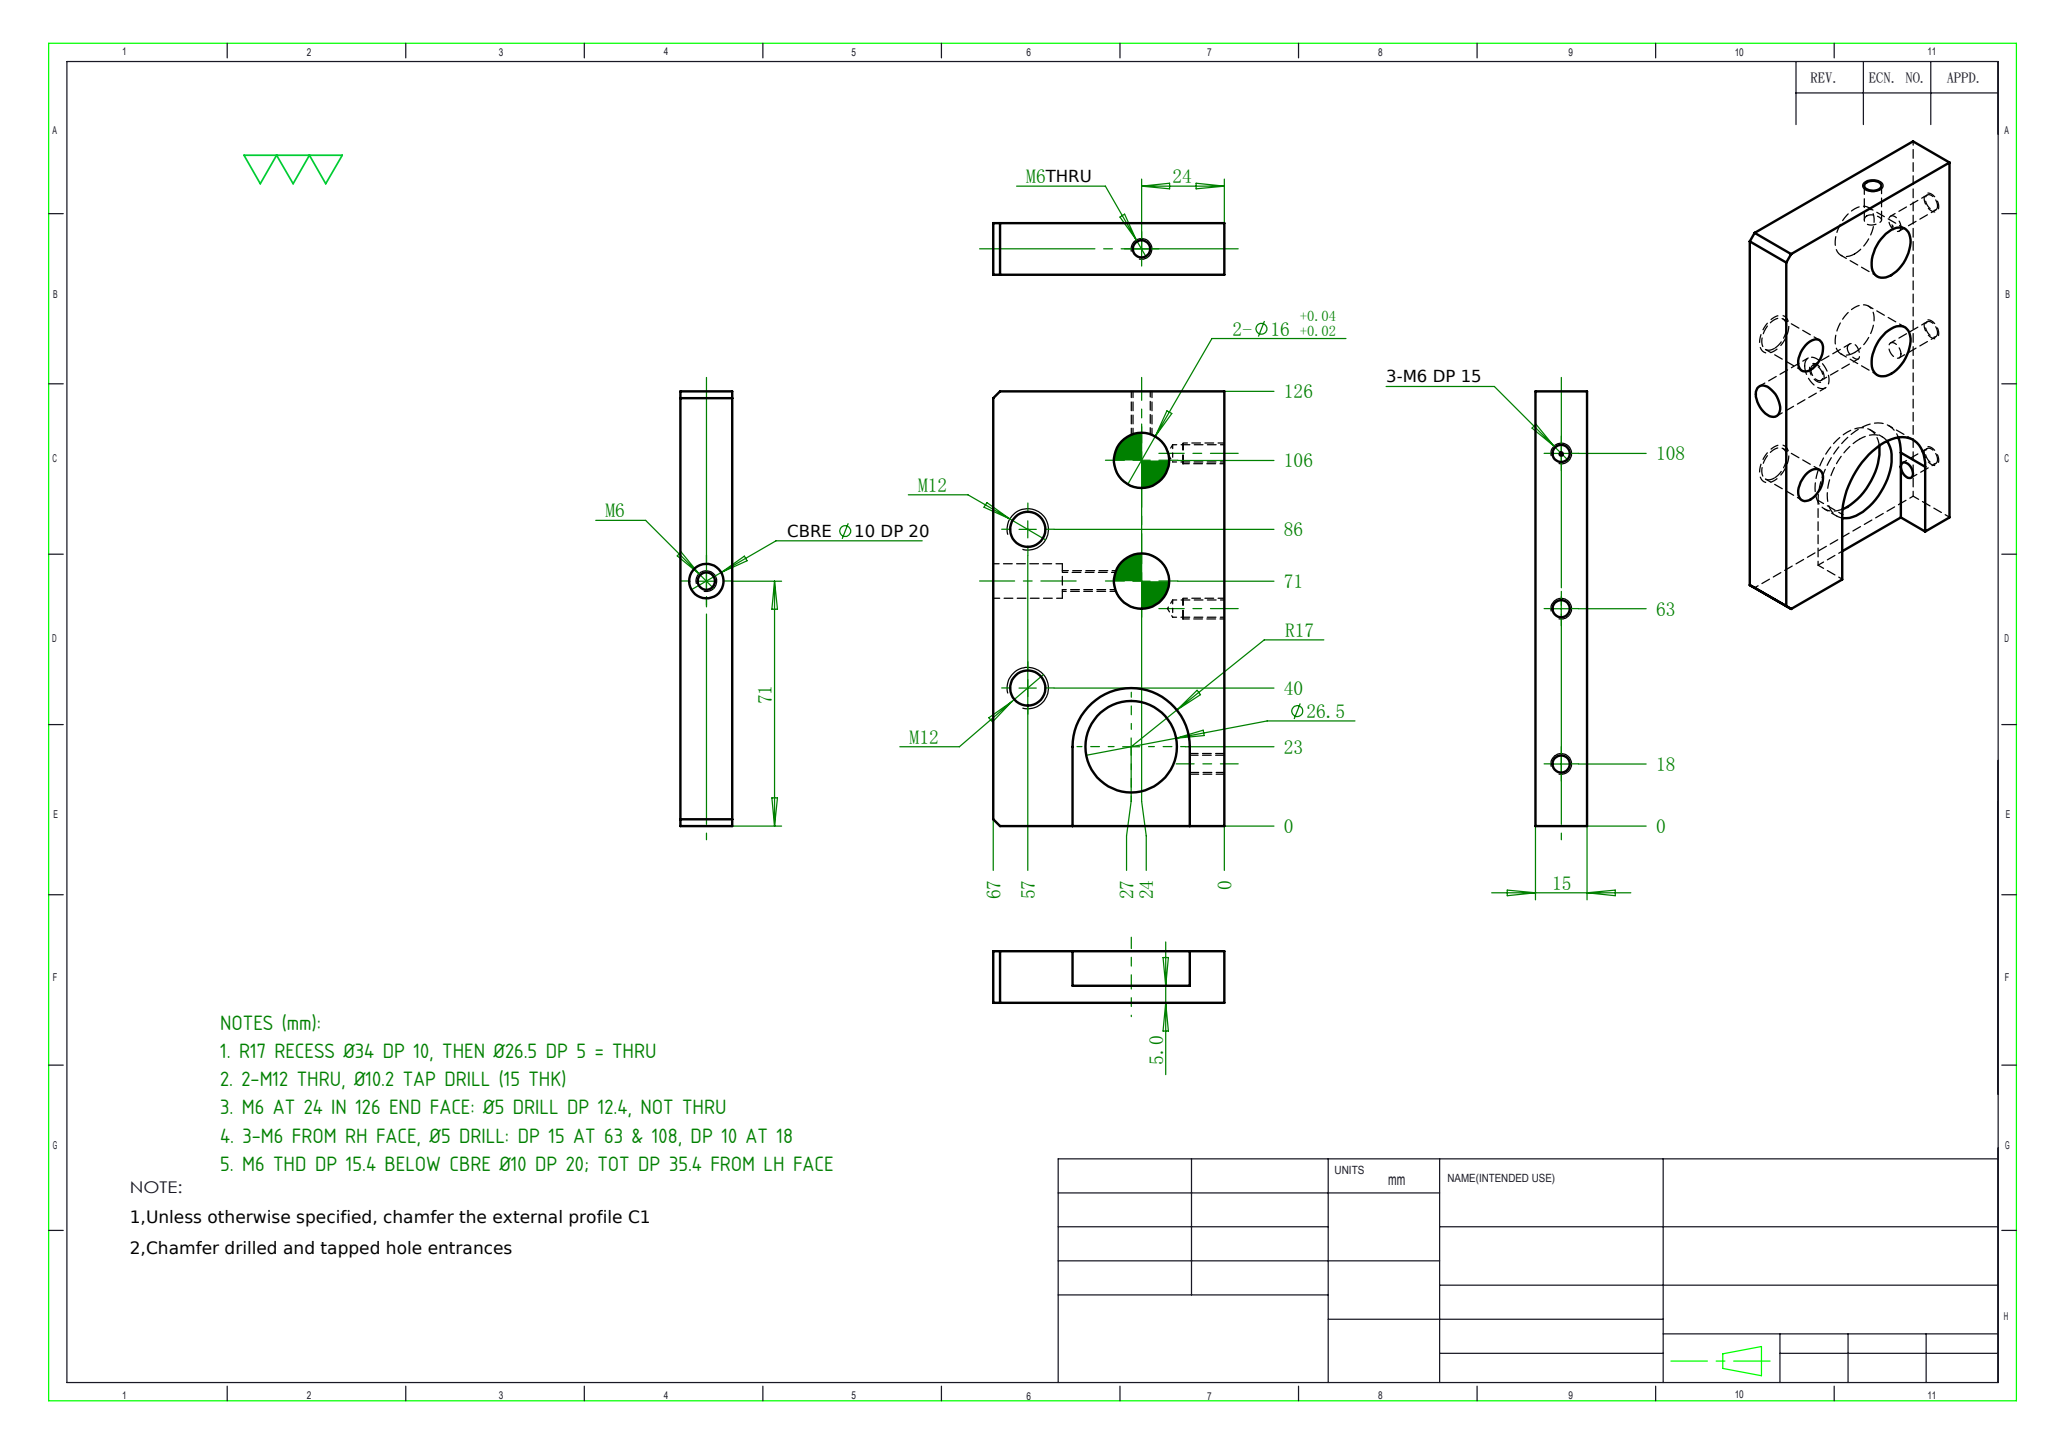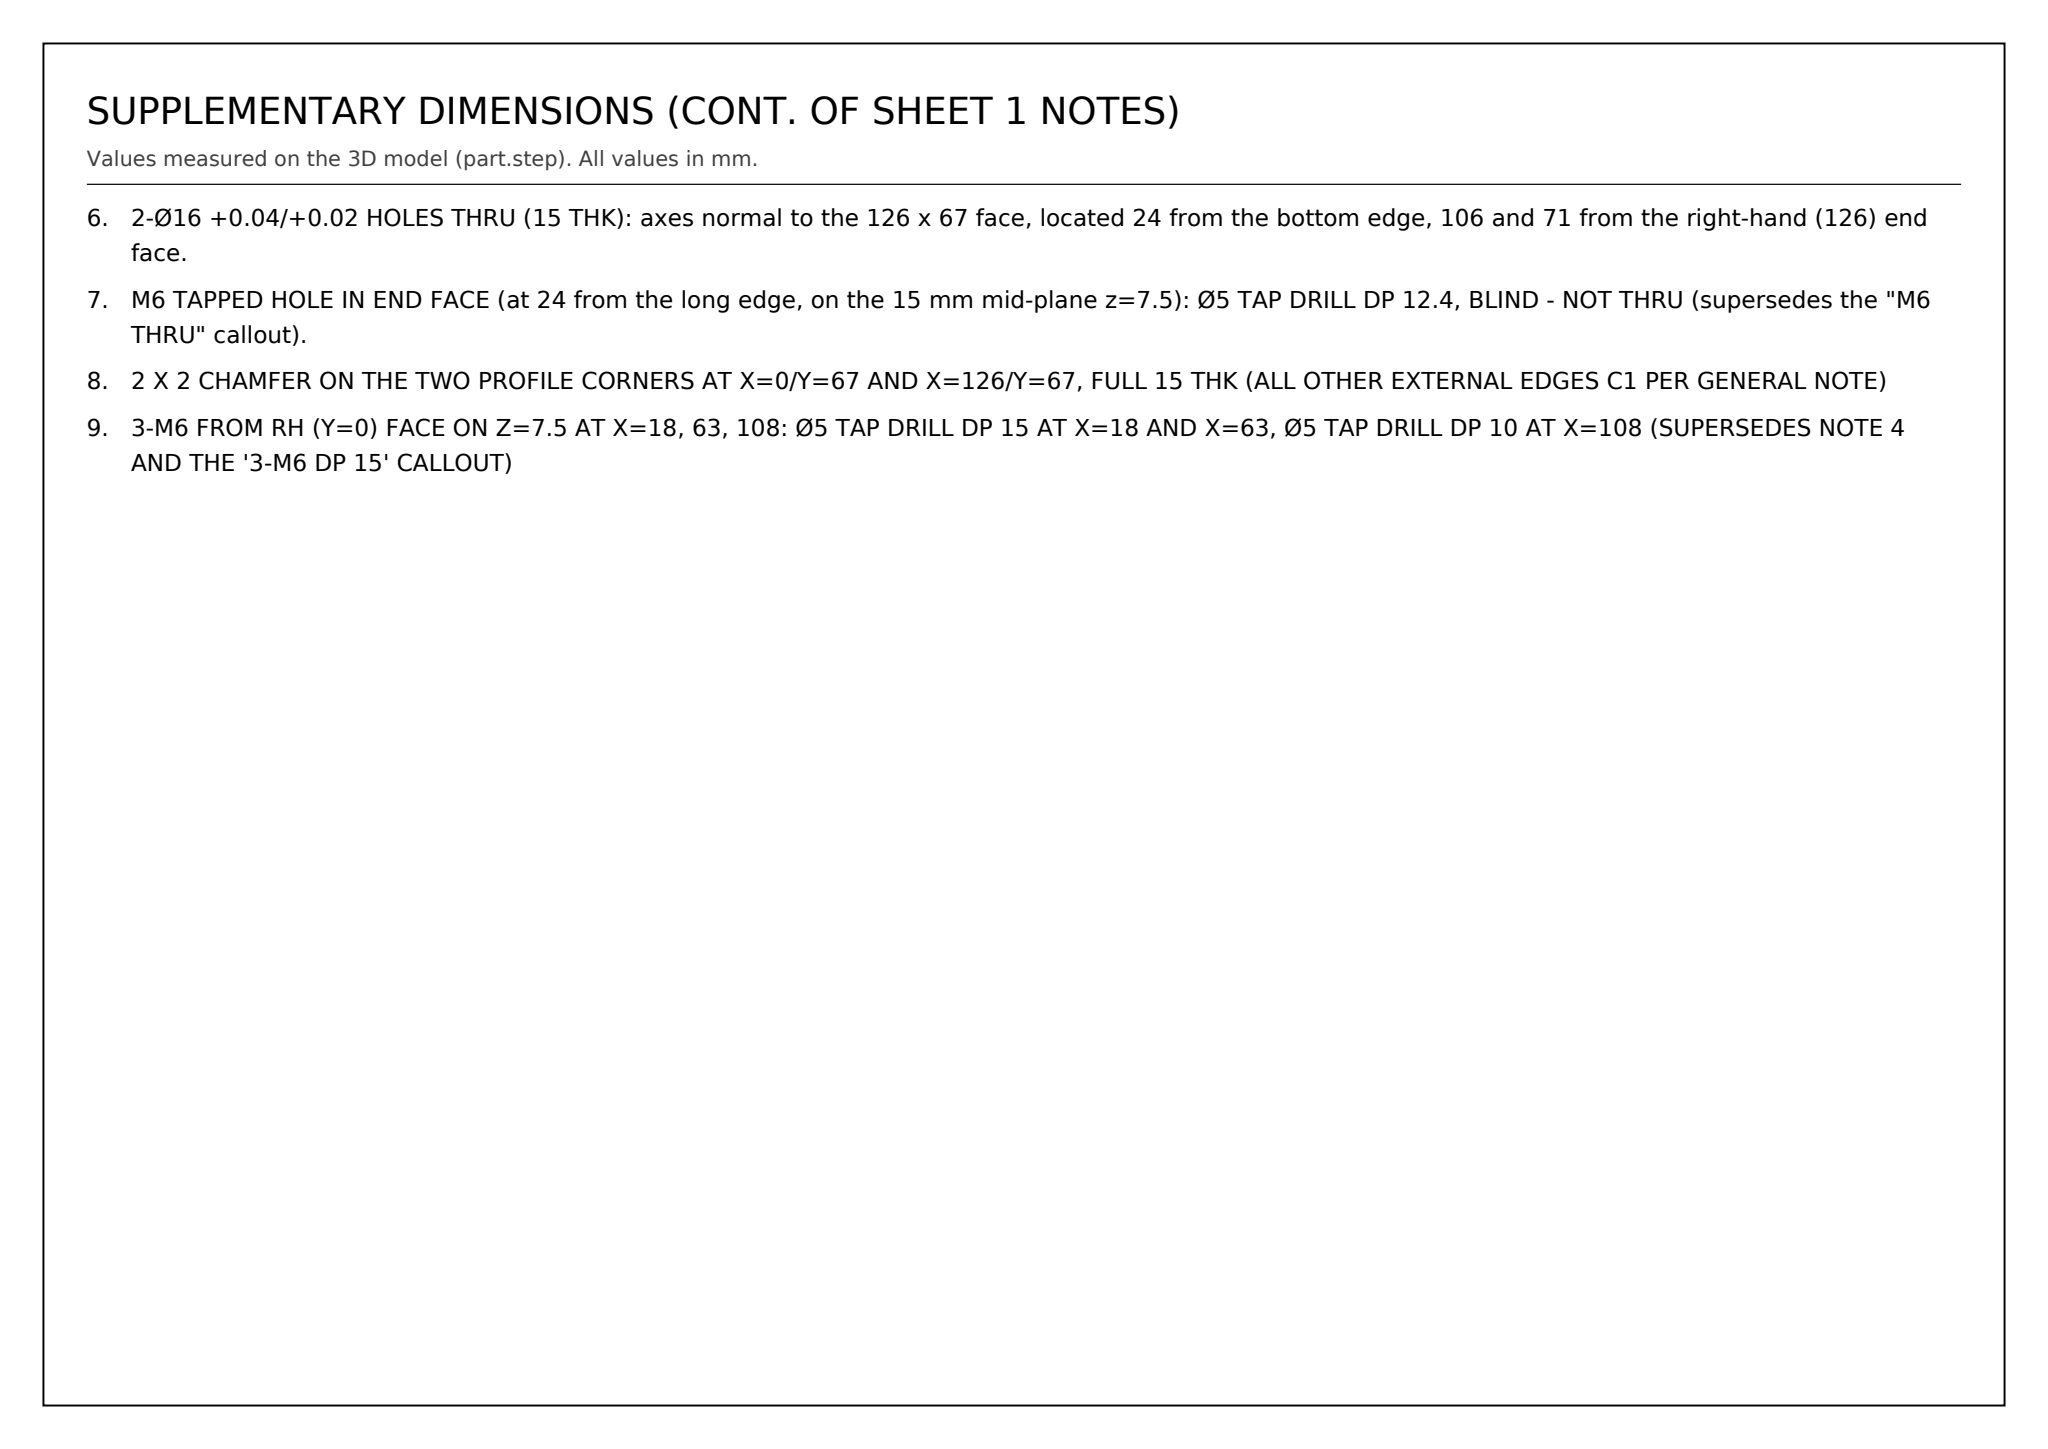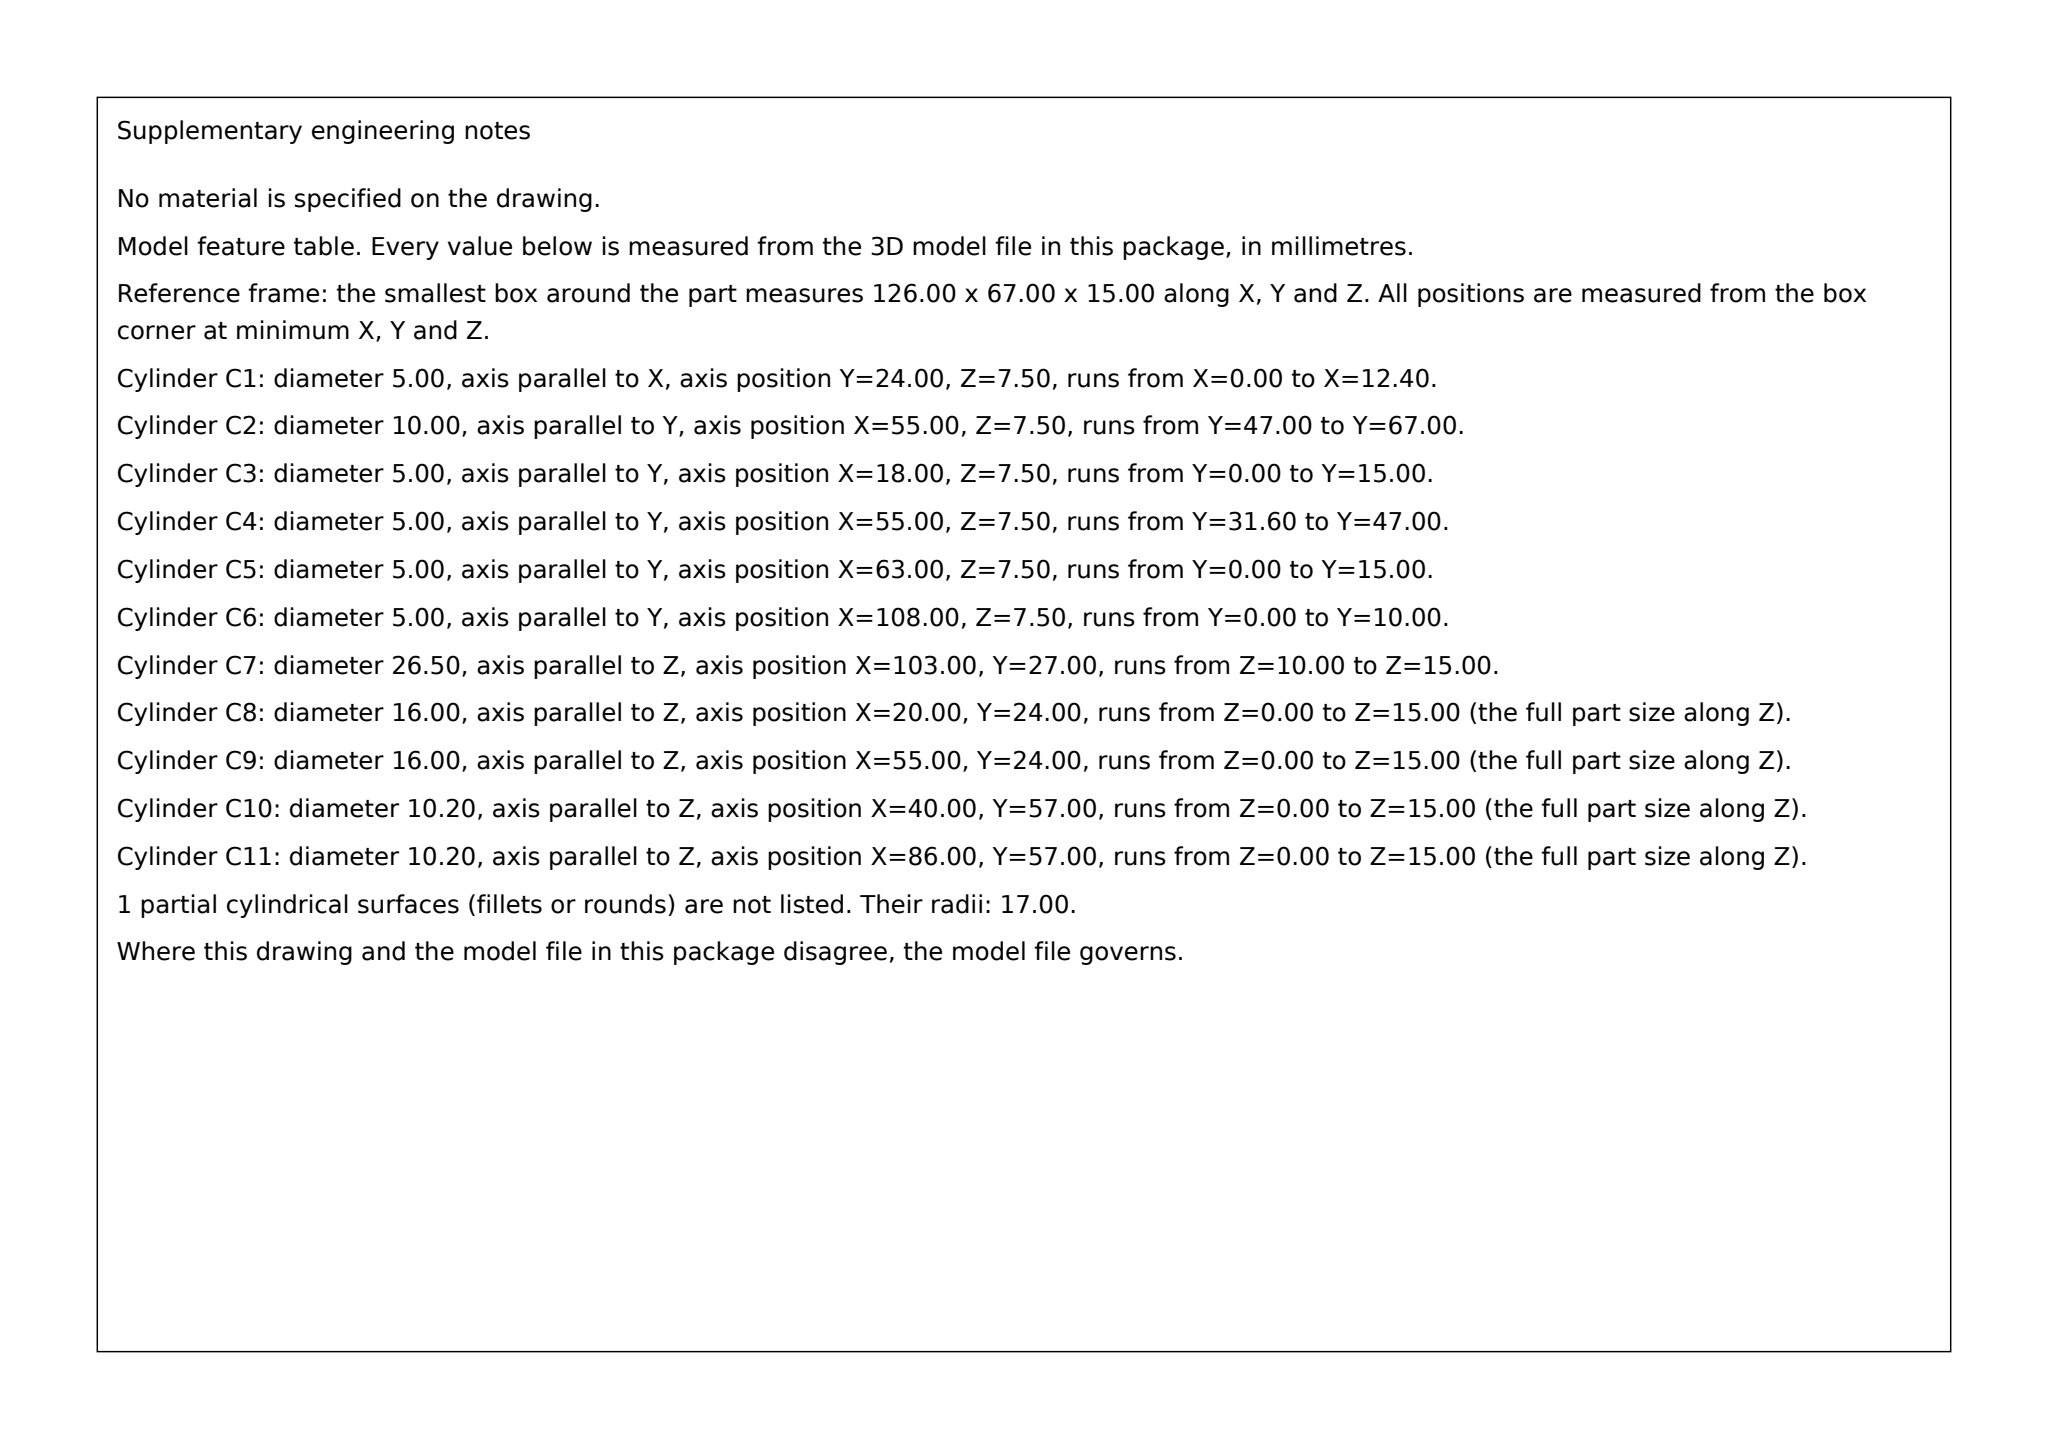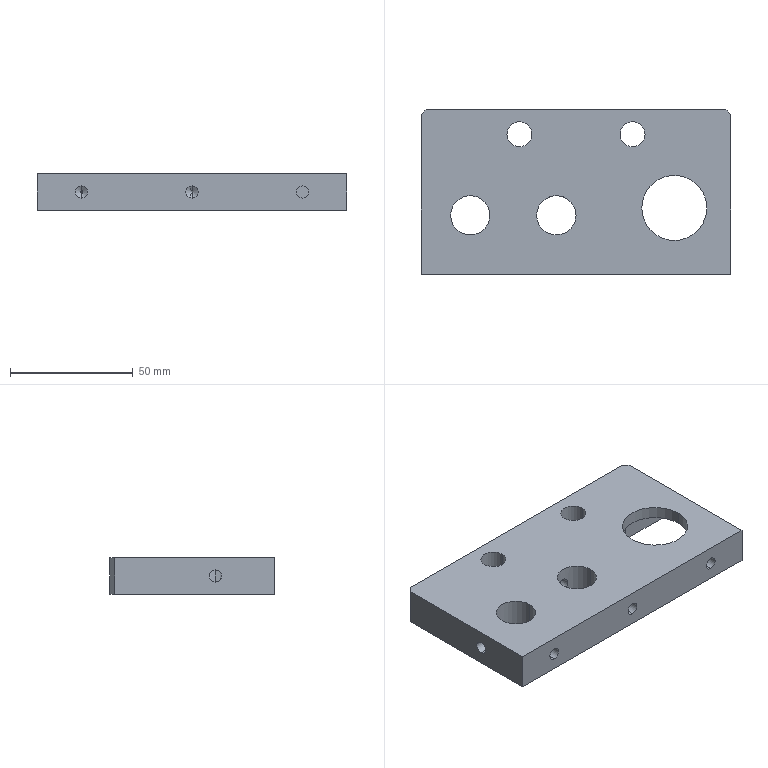Part | SolidWorks | mm | 1 solid | 40 faces | box 126 x 67 x 15 mm | volume 100060 mm3 | cylinder 24 | plane 12 | cone 4 | commonest cylinder face diameters 5 x10 16 x4 10.2 x4 10 x2 34 x2 26.5 x2
Drawing notes:
R17 RECESS Ø34 DP 10, THEN Ø26.5 DP 5 = THRU | from the solid: Ø34 z-cyl L=10 + Ø26.5 z-cyl L=5 at (103,27); z planes 0,10,15
2-M12 THRU, Ø10.2 TAP DRILL (15 THK) | from the solid: Ø10.2 z-cyls at (40,57) & (86,57), L=15 = thru plate
M6 AT 24 IN 126 END FACE: Ø5 DRILL DP 12.4, NOT THRU | from the solid: Ø5 x-axis cyl at y=24, z=7.5, L=12.4 from x=0 end; no thru bore
3-M6 FROM RH FACE, Ø5 DRILL: DP 15 AT 63 & 108, DP 10 AT 18 | from the solid: Ø5 y-cyls z=7.5: x=18 L=15 (dwg 108), x=63 L=15, x=108 L=10 (dwg 18)
M6 THD DP 15.4 BELOW CBRE Ø10 DP 20; TOT DP 35.4 FROM LH FACE | from the solid: y-axis cyls at x=55,z=7.5: Ø10 L20 c'bore (face y=67 to y=47 plane) + Ø5 L15.4 drill/tap below it; total 35.4
2-Ø16 +0.04/+0.02 HOLES THRU (15 THK): axes normal to the 126 x 67 face, located 24 from the bottom edge, 106 and 71 from the right-hand (126) end face. | from the solid: cylinders: hole/bore dia 16.0, axis z at [20.0,24.0] and [55.0,24.0], from 0.0 to 15.0 (plate thickness bbox z = 15.0)
M6 TAPPED HOLE IN END FACE (at 24 from the long edge, on the 15 mm mid-plane z=7.5): Ø5 TAP DRILL DP 12.4, BLIND - NOT THRU (supersedes the "M6 THRU" callout). | from the solid: cylinders: hole/bore dia 5.0, axis x at [y 24.0, z 7.5], from 0.0 to 12.4 (part length 126.0, so hole is blind)
2 X 2 CHAMFER ON THE TWO PROFILE CORNERS AT X=0/Y=67 AND X=126/Y=67, FULL 15 THK (ALL OTHER EXTERNAL EDGES C1 PER GENERAL NOTE) | from the solid: inclined_planes: two 45/45/90 faces, bbox_from [0,65,0] and [124,65,0], size [2,2,15]
3-M6 FROM RH (Y=0) FACE ON Z=7.5 AT X=18, 63, 108: Ø5 TAP DRILL DP 15 AT X=18 AND X=63, Ø5 TAP DRILL DP 10 AT X=108 (SUPERSEDES NOTE 4 AND THE '3-M6 DP 15' CALLOUT) | from the solid: cylinders: dia 5.0 axis y at x=18 from 0 to 15; dia 5.0 axis y at x=63 from 0 to 15; dia 5.0 axis y at x=108 from 0 to 10
build123d program:
from build123d import *

# Parameters (mm, degrees)
SKETCH1_W              = 126
SKETCH1_H              = 47
BOSS_EXTRUDE1_DEPTH    = 15
SKETCH2_R              = 13.25
CUT_EXTRUDE1_DEPTH     = 69.893
CUT_EXTRUDE2_DEPTH     = 10
SKETCH4_R              = 8
CUT_EXTRUDE3_DEPTH     = 69.893
SKETCH5_W              = 126
SKETCH5_H              = 15
BOSS_EXTRUDE2_DEPTH    = 20
M12_X1_TAPPED_HOLE1_D  = 10.2
M12_TAPPED_HOLE2_D     = 10.2
M6_TAPPED_HOLE1_REACH  = 136.139
M6_TAPPED_HOLE1_BORE_R = 2.5
CHAMFER1_SIZE          = 2
M6_TAPPED_HOLE2_D      = 5
M6_TAPPED_HOLE2_DEPTH  = 15
M6_TAPPED_HOLE2_TIP    = 1.502
LPATTERN1_COUNT        = 2
LPATTERN1_PITCH        = 35
M6_TAPPED_HOLE3_REACH  = 95.183
M6_TAPPED_HOLE3_BORE_R = 2.5
SKETCH19_R             = 5
CUT_EXTRUDE4_DEPTH     = 20


with BuildPart() as part:
    # Sketch1 → Boss-Extrude1 (new body)
    with BuildSketch(Plane.XY):
        Rectangle(SKETCH1_W, SKETCH1_H)
    extrude(amount=BOSS_EXTRUDE1_DEPTH)

    # Sketch2 → Cut-Extrude1 (cut, through all)
    with BuildSketch(Plane.XY.offset(15)):
        with Locations((40, 3.5)):
            Circle(SKETCH2_R)
    extrude(amount=-CUT_EXTRUDE1_DEPTH, mode=Mode.SUBTRACT)

    # Sketch3 → Cut-Extrude2 (cut)
    with BuildSketch(Plane(origin=(0, 0, 0), x_dir=(-1, 0, 0), z_dir=(0, 0, -1))):
        with BuildLine():
            Line((-40, -13.5), (-63, -13.5))
            ThreePointArc((-63, -13.5), (-80, 3.5), (-63, 20.5))
            Line((-63, 20.5), (-40, 20.5))
            ThreePointArc((-40, 20.5), (-23, 3.5), (-40, -13.5))
        make_face()
    extrude(amount=-CUT_EXTRUDE2_DEPTH, mode=Mode.SUBTRACT)

    # Sketch4 → Cut-Extrude3 (cut, through all)
    with BuildSketch(Plane.XY.offset(15)):
        with Locations((-43, 0.5)):
            Circle(SKETCH4_R)
    cut_extrude3 = extrude(amount=-CUT_EXTRUDE3_DEPTH, mode=Mode.SUBTRACT)

    # Sketch5 → Boss-Extrude2 (add)
    with BuildSketch(Plane(origin=(0, 23.5, 0), x_dir=(1, 0, 0), z_dir=(0, 1, 0))):
        with Locations((0, -7.5)):
            Rectangle(SKETCH5_W, SKETCH5_H)
    extrude(amount=BOSS_EXTRUDE2_DEPTH)

    # M12 x1 Tapped Hole1 (through all)
    with Locations(Plane.XY.offset(15)):
        with Locations((23, 33.5)):
            Hole(M12_X1_TAPPED_HOLE1_D / 2)

    # M12 Tapped Hole2 (through all)
    with Locations(Plane.XY.offset(15)):
        with Locations((-23, 33.5)):
            Hole(M12_TAPPED_HOLE2_D / 2)

    # M6 Tapped Hole1 bore → M6 Tapped Hole1 (cut, up to next)
    with BuildSketch(Plane.ZY.offset(63), mode=Mode.PRIVATE) as m6_tapped_hole1_sk1:
        with Locations((7.5, 0.5)):
            Circle(M6_TAPPED_HOLE1_BORE_R)
    m6_tapped_hole1_tool1 = extrude(m6_tapped_hole1_sk1.sketch, amount=-M6_TAPPED_HOLE1_REACH, mode=Mode.PRIVATE) & part.part
    add(m6_tapped_hole1_tool1.solids().sort_by_distance((-63, 0.5, 7.5))[0], mode=Mode.SUBTRACT)

    # Chamfer1
    chamfer1_edges = [part.edges().sort_by_distance(p)[0] for p in [
        (63, 43.5, 7.5),
        (-63, 43.5, 7.5),
    ]]
    chamfer(chamfer1_edges, length=CHAMFER1_SIZE)

    # M6 Tapped Hole2
    with Locations(Plane(origin=(0, -23.5, 0), x_dir=(-1, 0, 0), z_dir=(0, -1, 0))):
        with Locations((0, -7.5), (45, -7.5), (-45, -7.5)):
            Hole(M6_TAPPED_HOLE2_D / 2, depth=M6_TAPPED_HOLE2_DEPTH)
            with Locations((0, 0, -(M6_TAPPED_HOLE2_DEPTH + M6_TAPPED_HOLE2_TIP / 2))):  # 118° drill point
                Cone(0, M6_TAPPED_HOLE2_D / 2, M6_TAPPED_HOLE2_TIP, mode=Mode.SUBTRACT)

    # LPattern1: Cut-Extrude3 ×2
    with Locations(*[(i * LPATTERN1_PITCH, 0, 0) for i in range(1, LPATTERN1_COUNT)]):
        add(cut_extrude3, mode=Mode.SUBTRACT)

    # M6 Tapped Hole3 bore → M6 Tapped Hole3 (cut, up to next)
    with BuildSketch(Plane(origin=(0, 43.5, 0), x_dir=(1, 0, 0), z_dir=(0, 1, 0)), mode=Mode.PRIVATE) as m6_tapped_hole3_sk1:
        with Locations((-8, -7.5)):
            Circle(M6_TAPPED_HOLE3_BORE_R)
    m6_tapped_hole3_tool1 = extrude(m6_tapped_hole3_sk1.sketch, amount=-M6_TAPPED_HOLE3_REACH, mode=Mode.PRIVATE) & part.part
    add(m6_tapped_hole3_tool1.solids().sort_by_distance((-8, 43.5, 7.5))[0], mode=Mode.SUBTRACT)

    # Sketch19 → Cut-Extrude4 (cut)
    with BuildSketch(Plane(origin=(0, 43.5, 0), x_dir=(1, 0, 0), z_dir=(0, 1, 0))):
        with Locations(Location((-8, -7.5, 0), (0, 0, 270))):
            Circle(SKETCH19_R)
    extrude(amount=-CUT_EXTRUDE4_DEPTH, mode=Mode.SUBTRACT)


solid = part.part